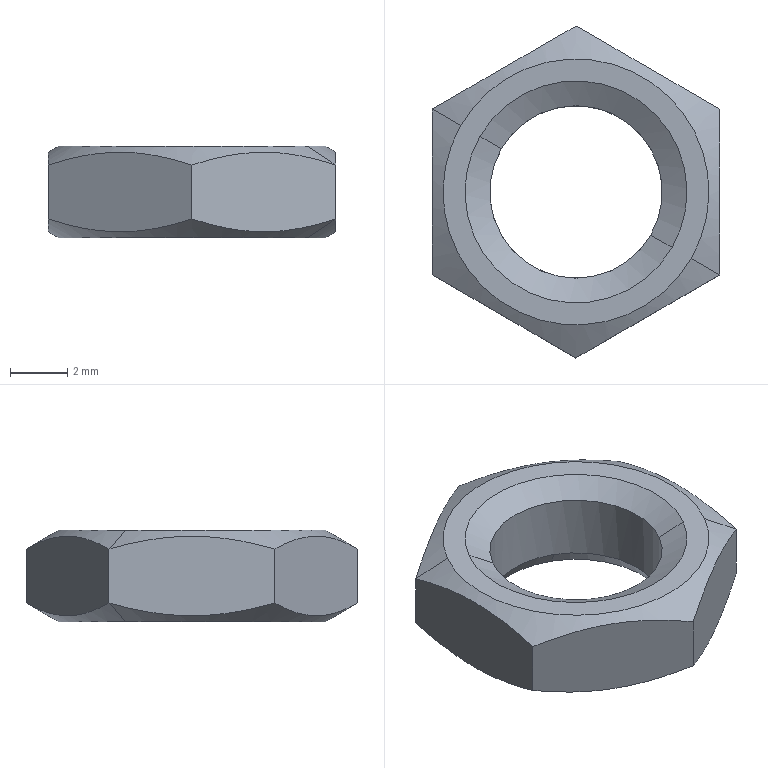Component | SolidWorks | HexThinNutGBT6172.1-M6-1 | 1 solid | 18 faces | box 10 x 11.55 x 3.2 mm | volume 173 mm3 | cone 8 | plane 8 | cylinder 2 | commonest cylinder face diameters 6 x2 | material Purchased Part
STEP:
#1=COLOUR_RGB('',0.7922,0.8196,0.9333);
#2=FILL_AREA_STYLE_COLOUR('',#1);
#3=FILL_AREA_STYLE('',(#2));
#4=SURFACE_STYLE_FILL_AREA(#3);
#5=SURFACE_SIDE_STYLE('',(#4));
#6=SURFACE_STYLE_USAGE(.BOTH.,#5);
#7=PRESENTATION_STYLE_ASSIGNMENT((#6));
#8=CARTESIAN_POINT('',(-1.968,-0.5242,-0.2756));
#9=VERTEX_POINT('',#8);
#10=CARTESIAN_POINT('',(-2.284,-0.3419,-0.2756));
#11=VERTEX_POINT('',#10);
#12=CARTESIAN_POINT('',(-2.126,-0.4331,-0.2756));
#13=DIRECTION('',(0.,0.,1.));
#14=DIRECTION('',(0.8657,-0.5005,0.));
#15=AXIS2_PLACEMENT_3D('',#12,#13,#14);
#16=CIRCLE('',#15,0.1821);
#17=EDGE_CURVE('',#9,#11,#16,.T.);
#18=ORIENTED_EDGE('',*,*,#17,.T.);
#19=CARTESIAN_POINT('',(-2.323,-0.3193,-0.2495));
#20=VERTEX_POINT('',#19);
#21=CARTESIAN_POINT('',(-2.323,-0.3192,-0.2493));
#22=DIRECTION('',(-0.7497,0.4335,0.5));
#23=VECTOR('',#22,39.37);
#24=LINE('',#21,#23);
#25=EDGE_CURVE('',#11,#20,#24,.T.);
#26=ORIENTED_EDGE('',*,*,#25,.T.);
#27=CARTESIAN_POINT('',(-2.126,-0.2058,-0.2495));
#28=VERTEX_POINT('',#27);
#29=CARTESIAN_POINT('',(-2.323,-0.3193,-0.2495));
#30=CARTESIAN_POINT('',(-2.291,-0.3008,-0.2602));
#31=CARTESIAN_POINT('',(-2.258,-0.2819,-0.267));
#32=CARTESIAN_POINT('',(-2.216,-0.2578,-0.2671));
#33=CARTESIAN_POINT('',(-2.208,-0.253,-0.2667));
#34=CARTESIAN_POINT('',(-2.191,-0.2434,-0.2651));
#35=CARTESIAN_POINT('',(-2.183,-0.2386,-0.2639));
#36=CARTESIAN_POINT('',(-2.158,-0.2244,-0.2593));
#37=CARTESIAN_POINT('',(-2.142,-0.215,-0.2548));
#38=CARTESIAN_POINT('',(-2.126,-0.2058,-0.2495));
#39=B_SPLINE_CURVE_WITH_KNOTS('',3,(#29,#30,#31,#32,#33,#34,#35,#36,#37,#38),.UNSPECIFIED.,.F.,.F.,(4,2,2,2,4),(0.,0.002915,0.003644,0.004373,0.005831),.UNSPECIFIED.);
#40=EDGE_CURVE('',#20,#28,#39,.T.);
#41=ORIENTED_EDGE('',*,*,#40,.T.);
#42=CARTESIAN_POINT('',(-1.929,-0.3195,-0.2495));
#43=VERTEX_POINT('',#42);
#44=CARTESIAN_POINT('',(-2.126,-0.2058,-0.2495));
#45=CARTESIAN_POINT('',(-2.094,-0.2243,-0.2602));
#46=CARTESIAN_POINT('',(-2.061,-0.2432,-0.267));
#47=CARTESIAN_POINT('',(-2.019,-0.2674,-0.2671));
#48=CARTESIAN_POINT('',(-2.011,-0.2722,-0.2667));
#49=CARTESIAN_POINT('',(-1.994,-0.2819,-0.2651));
#50=CARTESIAN_POINT('',(-1.986,-0.2866,-0.2639));
#51=CARTESIAN_POINT('',(-1.961,-0.3009,-0.2593));
#52=CARTESIAN_POINT('',(-1.945,-0.3102,-0.2548));
#53=CARTESIAN_POINT('',(-1.929,-0.3195,-0.2495));
#54=B_SPLINE_CURVE_WITH_KNOTS('',3,(#44,#45,#46,#47,#48,#49,#50,#51,#52,#53),.UNSPECIFIED.,.F.,.F.,(4,2,2,2,4),(0.,0.002915,0.003644,0.004373,0.005831),.UNSPECIFIED.);
#55=EDGE_CURVE('',#28,#43,#54,.T.);
#56=ORIENTED_EDGE('',*,*,#55,.T.);
#57=CARTESIAN_POINT('',(-1.929,-0.5468,-0.2495));
#58=VERTEX_POINT('',#57);
#59=CARTESIAN_POINT('',(-1.929,-0.3195,-0.2495));
#60=CARTESIAN_POINT('',(-1.929,-0.3567,-0.2602));
#61=CARTESIAN_POINT('',(-1.929,-0.3943,-0.267));
#62=CARTESIAN_POINT('',(-1.929,-0.4426,-0.2671));
#63=CARTESIAN_POINT('',(-1.929,-0.4523,-0.2667));
#64=CARTESIAN_POINT('',(-1.929,-0.4715,-0.2651));
#65=CARTESIAN_POINT('',(-1.929,-0.4811,-0.2639));
#66=CARTESIAN_POINT('',(-1.929,-0.5095,-0.2593));
#67=CARTESIAN_POINT('',(-1.929,-0.5283,-0.2548));
#68=CARTESIAN_POINT('',(-1.929,-0.5468,-0.2495));
#69=B_SPLINE_CURVE_WITH_KNOTS('',3,(#59,#60,#61,#62,#63,#64,#65,#66,#67,#68),.UNSPECIFIED.,.F.,.F.,(4,2,2,2,4),(0.,0.002915,0.003644,0.004373,0.005831),.UNSPECIFIED.);
#70=EDGE_CURVE('',#43,#58,#69,.T.);
#71=ORIENTED_EDGE('',*,*,#70,.T.);
#72=CARTESIAN_POINT('',(-1.929,-0.547,-0.2493));
#73=DIRECTION('',(0.7497,-0.4335,0.5));
#74=VECTOR('',#73,39.37);
#75=LINE('',#72,#74);
#76=EDGE_CURVE('',#9,#58,#75,.T.);
#77=ORIENTED_EDGE('',*,*,#76,.F.);
#78=EDGE_LOOP('',(#18,#26,#41,#56,#71,#77));
#79=FACE_OUTER_BOUND('',#78,.T.);
#80=CARTESIAN_POINT('',(-2.126,-0.4331,-0.2493));
#81=DIRECTION('',(0.,0.,1.));
#82=DIRECTION('',(0.8657,-0.5005,0.));
#83=AXIS2_PLACEMENT_3D('',#80,#81,#82);
#84=CONICAL_SURFACE('',#83,0.2276,1.047);
#85=ADVANCED_FACE('',(#79),#84,.T.);
#86=CARTESIAN_POINT('',(-2.185,-0.5353,-0.2573));
#87=VERTEX_POINT('',#86);
#88=CARTESIAN_POINT('',(-2.228,-0.374,-0.2573));
#89=VERTEX_POINT('',#88);
#90=CARTESIAN_POINT('',(-2.126,-0.4331,-0.2573));
#91=DIRECTION('',(0.,0.,-1.));
#92=DIRECTION('',(0.5005,0.8657,0.));
#93=AXIS2_PLACEMENT_3D('',#90,#91,#92);
#94=CIRCLE('',#93,0.1181);
#95=EDGE_CURVE('',#87,#89,#94,.T.);
#96=ORIENTED_EDGE('',*,*,#95,.F.);
#97=CARTESIAN_POINT('',(-2.19,-0.5445,-0.2756));
#98=VERTEX_POINT('',#97);
#99=CARTESIAN_POINT('',(-2.187,-0.5391,-0.2649));
#100=DIRECTION('',(-0.2503,-0.4329,-0.866));
#101=VECTOR('',#100,39.37);
#102=LINE('',#99,#101);
#103=EDGE_CURVE('',#87,#98,#102,.T.);
#104=ORIENTED_EDGE('',*,*,#103,.T.);
#105=CARTESIAN_POINT('',(-2.062,-0.3217,-0.2756));
#106=VERTEX_POINT('',#105);
#107=CARTESIAN_POINT('',(-2.126,-0.4331,-0.2756));
#108=DIRECTION('',(0.,0.,-1.));
#109=DIRECTION('',(0.8657,-0.5005,0.));
#110=AXIS2_PLACEMENT_3D('',#107,#108,#109);
#111=CIRCLE('',#110,0.1287);
#112=EDGE_CURVE('',#98,#106,#111,.T.);
#113=ORIENTED_EDGE('',*,*,#112,.T.);
#114=CARTESIAN_POINT('',(-2.067,-0.3308,-0.2573));
#115=VERTEX_POINT('',#114);
#116=CARTESIAN_POINT('',(-2.065,-0.327,-0.2649));
#117=DIRECTION('',(0.2503,0.4329,-0.866));
#118=VECTOR('',#117,39.37);
#119=LINE('',#116,#118);
#120=EDGE_CURVE('',#115,#106,#119,.T.);
#121=ORIENTED_EDGE('',*,*,#120,.F.);
#122=CARTESIAN_POINT('',(-2.126,-0.4331,-0.2573));
#123=DIRECTION('',(0.,0.,-1.));
#124=DIRECTION('',(0.5005,0.8657,0.));
#125=AXIS2_PLACEMENT_3D('',#122,#123,#124);
#126=CIRCLE('',#125,0.1181);
#127=EDGE_CURVE('',#89,#115,#126,.T.);
#128=ORIENTED_EDGE('',*,*,#127,.F.);
#129=EDGE_LOOP('',(#96,#104,#113,#121,#128));
#130=FACE_OUTER_BOUND('',#129,.T.);
#131=CARTESIAN_POINT('',(-2.126,-0.4331,-0.2649));
#132=DIRECTION('',(0.,0.,-1.));
#133=DIRECTION('',(0.5005,0.8657,0.));
#134=AXIS2_PLACEMENT_3D('',#131,#132,#133);
#135=CONICAL_SURFACE('',#134,0.1225,0.5236);
#136=ADVANCED_FACE('',(#130),#135,.F.);
#137=CARTESIAN_POINT('',(-2.024,-0.4922,-0.2573));
#138=VERTEX_POINT('',#137);
#139=CARTESIAN_POINT('',(-2.126,-0.4331,-0.2573));
#140=DIRECTION('',(0.,0.,-1.));
#141=DIRECTION('',(0.5005,0.8657,0.));
#142=AXIS2_PLACEMENT_3D('',#139,#140,#141);
#143=CIRCLE('',#142,0.1181);
#144=EDGE_CURVE('',#138,#87,#143,.T.);
#145=ORIENTED_EDGE('',*,*,#144,.T.);
#146=ORIENTED_EDGE('',*,*,#95,.T.);
#147=CARTESIAN_POINT('',(-2.228,-0.374,-0.1692));
#148=VERTEX_POINT('',#147);
#149=CARTESIAN_POINT('',(-2.228,-0.374,-0.2756));
#150=DIRECTION('',(0.,0.,1.));
#151=VECTOR('',#150,39.37);
#152=LINE('',#149,#151);
#153=EDGE_CURVE('',#89,#148,#152,.T.);
#154=ORIENTED_EDGE('',*,*,#153,.T.);
#155=CARTESIAN_POINT('',(-2.024,-0.4922,-0.1692));
#156=VERTEX_POINT('',#155);
#157=CARTESIAN_POINT('',(-2.126,-0.4331,-0.1692));
#158=DIRECTION('',(0.,0.,-1.));
#159=DIRECTION('',(0.8657,-0.5005,0.));
#160=AXIS2_PLACEMENT_3D('',#157,#158,#159);
#161=CIRCLE('',#160,0.1181);
#162=EDGE_CURVE('',#156,#148,#161,.T.);
#163=ORIENTED_EDGE('',*,*,#162,.F.);
#164=CARTESIAN_POINT('',(-2.024,-0.4922,-0.2756));
#165=DIRECTION('',(0.,0.,1.));
#166=VECTOR('',#165,39.37);
#167=LINE('',#164,#166);
#168=EDGE_CURVE('',#138,#156,#167,.T.);
#169=ORIENTED_EDGE('',*,*,#168,.F.);
#170=EDGE_LOOP('',(#145,#146,#154,#163,#169));
#171=FACE_OUTER_BOUND('',#170,.T.);
#172=CARTESIAN_POINT('',(-2.126,-0.4331,-0.2756));
#173=DIRECTION('',(0.,0.,1.));
#174=DIRECTION('',(0.8657,-0.5005,0.));
#175=AXIS2_PLACEMENT_3D('',#172,#173,#174);
#176=CYLINDRICAL_SURFACE('',#175,0.1181);
#177=ADVANCED_FACE('',(#171),#176,.F.);
#178=CARTESIAN_POINT('',(-2.284,-0.3419,-0.1496));
#179=VERTEX_POINT('',#178);
#180=CARTESIAN_POINT('',(-1.968,-0.5242,-0.1496));
#181=VERTEX_POINT('',#180);
#182=CARTESIAN_POINT('',(-2.126,-0.4331,-0.1496));
#183=DIRECTION('',(0.,0.,-1.));
#184=DIRECTION('',(-0.8657,0.5005,0.));
#185=AXIS2_PLACEMENT_3D('',#182,#183,#184);
#186=CIRCLE('',#185,0.1821);
#187=EDGE_CURVE('',#179,#181,#186,.T.);
#188=ORIENTED_EDGE('',*,*,#187,.T.);
#189=CARTESIAN_POINT('',(-1.929,-0.5468,-0.1757));
#190=VERTEX_POINT('',#189);
#191=CARTESIAN_POINT('',(-1.929,-0.547,-0.1759));
#192=DIRECTION('',(0.7497,-0.4335,-0.5));
#193=VECTOR('',#192,39.37);
#194=LINE('',#191,#193);
#195=EDGE_CURVE('',#181,#190,#194,.T.);
#196=ORIENTED_EDGE('',*,*,#195,.T.);
#197=CARTESIAN_POINT('',(-1.929,-0.3195,-0.1757));
#198=VERTEX_POINT('',#197);
#199=CARTESIAN_POINT('',(-1.929,-0.3195,-0.1757));
#200=CARTESIAN_POINT('',(-1.929,-0.3567,-0.165));
#201=CARTESIAN_POINT('',(-1.929,-0.3943,-0.1582));
#202=CARTESIAN_POINT('',(-1.929,-0.4426,-0.1581));
#203=CARTESIAN_POINT('',(-1.929,-0.4523,-0.1585));
#204=CARTESIAN_POINT('',(-1.929,-0.4715,-0.1601));
#205=CARTESIAN_POINT('',(-1.929,-0.4811,-0.1613));
#206=CARTESIAN_POINT('',(-1.929,-0.5095,-0.1659));
#207=CARTESIAN_POINT('',(-1.929,-0.5283,-0.1703));
#208=CARTESIAN_POINT('',(-1.929,-0.5468,-0.1757));
#209=B_SPLINE_CURVE_WITH_KNOTS('',3,(#199,#200,#201,#202,#203,#204,#205,#206,#207,#208),.UNSPECIFIED.,.F.,.F.,(4,2,2,2,4),(0.,0.002915,0.003644,0.004373,0.005831),.UNSPECIFIED.);
#210=EDGE_CURVE('',#198,#190,#209,.T.);
#211=ORIENTED_EDGE('',*,*,#210,.F.);
#212=CARTESIAN_POINT('',(-2.126,-0.2058,-0.1757));
#213=VERTEX_POINT('',#212);
#214=CARTESIAN_POINT('',(-2.126,-0.2058,-0.1757));
#215=CARTESIAN_POINT('',(-2.094,-0.2243,-0.165));
#216=CARTESIAN_POINT('',(-2.061,-0.2432,-0.1582));
#217=CARTESIAN_POINT('',(-2.019,-0.2674,-0.1581));
#218=CARTESIAN_POINT('',(-2.011,-0.2722,-0.1585));
#219=CARTESIAN_POINT('',(-1.994,-0.2819,-0.1601));
#220=CARTESIAN_POINT('',(-1.986,-0.2866,-0.1613));
#221=CARTESIAN_POINT('',(-1.961,-0.3009,-0.1659));
#222=CARTESIAN_POINT('',(-1.945,-0.3102,-0.1703));
#223=CARTESIAN_POINT('',(-1.929,-0.3195,-0.1757));
#224=B_SPLINE_CURVE_WITH_KNOTS('',3,(#214,#215,#216,#217,#218,#219,#220,#221,#222,#223),.UNSPECIFIED.,.F.,.F.,(4,2,2,2,4),(0.,0.002915,0.003644,0.004373,0.005831),.UNSPECIFIED.);
#225=EDGE_CURVE('',#213,#198,#224,.T.);
#226=ORIENTED_EDGE('',*,*,#225,.F.);
#227=CARTESIAN_POINT('',(-2.323,-0.3193,-0.1757));
#228=VERTEX_POINT('',#227);
#229=CARTESIAN_POINT('',(-2.323,-0.3193,-0.1757));
#230=CARTESIAN_POINT('',(-2.291,-0.3008,-0.165));
#231=CARTESIAN_POINT('',(-2.258,-0.2819,-0.1582));
#232=CARTESIAN_POINT('',(-2.216,-0.2578,-0.1581));
#233=CARTESIAN_POINT('',(-2.208,-0.253,-0.1585));
#234=CARTESIAN_POINT('',(-2.191,-0.2434,-0.1601));
#235=CARTESIAN_POINT('',(-2.183,-0.2386,-0.1613));
#236=CARTESIAN_POINT('',(-2.158,-0.2244,-0.1659));
#237=CARTESIAN_POINT('',(-2.142,-0.215,-0.1703));
#238=CARTESIAN_POINT('',(-2.126,-0.2058,-0.1757));
#239=B_SPLINE_CURVE_WITH_KNOTS('',3,(#229,#230,#231,#232,#233,#234,#235,#236,#237,#238),.UNSPECIFIED.,.F.,.F.,(4,2,2,2,4),(0.,0.002915,0.003644,0.004373,0.005831),.UNSPECIFIED.);
#240=EDGE_CURVE('',#228,#213,#239,.T.);
#241=ORIENTED_EDGE('',*,*,#240,.F.);
#242=CARTESIAN_POINT('',(-2.323,-0.3192,-0.1759));
#243=DIRECTION('',(-0.7497,0.4335,-0.5));
#244=VECTOR('',#243,39.37);
#245=LINE('',#242,#244);
#246=EDGE_CURVE('',#179,#228,#245,.T.);
#247=ORIENTED_EDGE('',*,*,#246,.F.);
#248=EDGE_LOOP('',(#188,#196,#211,#226,#241,#247));
#249=FACE_OUTER_BOUND('',#248,.T.);
#250=CARTESIAN_POINT('',(-2.126,-0.4331,-0.1759));
#251=DIRECTION('',(0.,0.,-1.));
#252=DIRECTION('',(-0.8657,0.5005,0.));
#253=AXIS2_PLACEMENT_3D('',#250,#251,#252);
#254=CONICAL_SURFACE('',#253,0.2276,1.047);
#255=ADVANCED_FACE('',(#249),#254,.T.);
#256=ORIENTED_EDGE('',*,*,#162,.T.);
#257=CARTESIAN_POINT('',(-2.258,-0.357,-0.1496));
#258=VERTEX_POINT('',#257);
#259=CARTESIAN_POINT('',(-2.23,-0.373,-0.1681));
#260=DIRECTION('',(-0.7497,0.4335,0.5));
#261=VECTOR('',#260,39.37);
#262=LINE('',#259,#261);
#263=EDGE_CURVE('',#148,#258,#262,.T.);
#264=ORIENTED_EDGE('',*,*,#263,.T.);
#265=CARTESIAN_POINT('',(-1.994,-0.5092,-0.1496));
#266=VERTEX_POINT('',#265);
#267=CARTESIAN_POINT('',(-2.126,-0.4331,-0.1496));
#268=DIRECTION('',(0.,0.,-1.));
#269=DIRECTION('',(0.8657,-0.5005,0.));
#270=AXIS2_PLACEMENT_3D('',#267,#268,#269);
#271=CIRCLE('',#270,0.152);
#272=EDGE_CURVE('',#266,#258,#271,.T.);
#273=ORIENTED_EDGE('',*,*,#272,.F.);
#274=CARTESIAN_POINT('',(-2.022,-0.4932,-0.1681));
#275=DIRECTION('',(0.7497,-0.4335,0.5));
#276=VECTOR('',#275,39.37);
#277=LINE('',#274,#276);
#278=EDGE_CURVE('',#156,#266,#277,.T.);
#279=ORIENTED_EDGE('',*,*,#278,.F.);
#280=EDGE_LOOP('',(#256,#264,#273,#279));
#281=FACE_OUTER_BOUND('',#280,.T.);
#282=CARTESIAN_POINT('',(-2.126,-0.4331,-0.1681));
#283=DIRECTION('',(0.,0.,1.));
#284=DIRECTION('',(0.8657,-0.5005,0.));
#285=AXIS2_PLACEMENT_3D('',#282,#283,#284);
#286=CONICAL_SURFACE('',#285,0.12,1.047);
#287=ADVANCED_FACE('',(#281),#286,.F.);
#288=ORIENTED_EDGE('',*,*,#17,.F.);
#289=CARTESIAN_POINT('',(-2.126,-0.4331,-0.2756));
#290=DIRECTION('',(0.,0.,1.));
#291=DIRECTION('',(0.8657,-0.5005,0.));
#292=AXIS2_PLACEMENT_3D('',#289,#290,#291);
#293=CIRCLE('',#292,0.1821);
#294=EDGE_CURVE('',#11,#9,#293,.T.);
#295=ORIENTED_EDGE('',*,*,#294,.F.);
#296=EDGE_LOOP('',(#288,#295));
#297=FACE_OUTER_BOUND('',#296,.T.);
#298=CARTESIAN_POINT('',(-2.126,-0.4331,-0.2756));
#299=DIRECTION('',(0.,0.,-1.));
#300=DIRECTION('',(0.8657,-0.5005,0.));
#301=AXIS2_PLACEMENT_3D('',#298,#299,#300);
#302=CIRCLE('',#301,0.1287);
#303=EDGE_CURVE('',#106,#98,#302,.T.);
#304=ORIENTED_EDGE('',*,*,#303,.F.);
#305=ORIENTED_EDGE('',*,*,#112,.F.);
#306=EDGE_LOOP('',(#304,#305));
#307=FACE_BOUND('',#306,.T.);
#308=CARTESIAN_POINT('',(-2.126,-0.6604,-0.2756));
#309=DIRECTION('',(0.,0.,1.));
#310=DIRECTION('',(0.8657,-0.5005,0.));
#311=AXIS2_PLACEMENT_3D('',#308,#309,#310);
#312=PLANE('',#311);
#313=ADVANCED_FACE('',(#297,#307),#312,.F.);
#314=ORIENTED_EDGE('',*,*,#25,.F.);
#315=ORIENTED_EDGE('',*,*,#294,.T.);
#316=ORIENTED_EDGE('',*,*,#76,.T.);
#317=CARTESIAN_POINT('',(-2.126,-0.6604,-0.2495));
#318=VERTEX_POINT('',#317);
#319=CARTESIAN_POINT('',(-1.929,-0.5468,-0.2495));
#320=CARTESIAN_POINT('',(-1.961,-0.5654,-0.2602));
#321=CARTESIAN_POINT('',(-1.994,-0.5842,-0.267));
#322=CARTESIAN_POINT('',(-2.036,-0.6083,-0.2671));
#323=CARTESIAN_POINT('',(-2.044,-0.6132,-0.2667));
#324=CARTESIAN_POINT('',(-2.061,-0.6228,-0.2651));
#325=CARTESIAN_POINT('',(-2.069,-0.6275,-0.2639));
#326=CARTESIAN_POINT('',(-2.094,-0.6417,-0.2593));
#327=CARTESIAN_POINT('',(-2.11,-0.6511,-0.2548));
#328=CARTESIAN_POINT('',(-2.126,-0.6604,-0.2495));
#329=B_SPLINE_CURVE_WITH_KNOTS('',3,(#319,#320,#321,#322,#323,#324,#325,#326,#327,#328),.UNSPECIFIED.,.F.,.F.,(4,2,2,2,4),(0.,0.002915,0.003644,0.004373,0.005831),.UNSPECIFIED.);
#330=EDGE_CURVE('',#58,#318,#329,.T.);
#331=ORIENTED_EDGE('',*,*,#330,.T.);
#332=CARTESIAN_POINT('',(-2.323,-0.5466,-0.2495));
#333=VERTEX_POINT('',#332);
#334=CARTESIAN_POINT('',(-2.126,-0.6604,-0.2495));
#335=CARTESIAN_POINT('',(-2.158,-0.6418,-0.2602));
#336=CARTESIAN_POINT('',(-2.191,-0.6229,-0.267));
#337=CARTESIAN_POINT('',(-2.233,-0.5988,-0.2671));
#338=CARTESIAN_POINT('',(-2.241,-0.5939,-0.2667));
#339=CARTESIAN_POINT('',(-2.258,-0.5843,-0.2651));
#340=CARTESIAN_POINT('',(-2.266,-0.5795,-0.2639));
#341=CARTESIAN_POINT('',(-2.291,-0.5653,-0.2593));
#342=CARTESIAN_POINT('',(-2.307,-0.5559,-0.2548));
#343=CARTESIAN_POINT('',(-2.323,-0.5466,-0.2495));
#344=B_SPLINE_CURVE_WITH_KNOTS('',3,(#334,#335,#336,#337,#338,#339,#340,#341,#342,#343),.UNSPECIFIED.,.F.,.F.,(4,2,2,2,4),(0.,0.002915,0.003644,0.004373,0.005831),.UNSPECIFIED.);
#345=EDGE_CURVE('',#318,#333,#344,.T.);
#346=ORIENTED_EDGE('',*,*,#345,.T.);
#347=CARTESIAN_POINT('',(-2.323,-0.5466,-0.2495));
#348=CARTESIAN_POINT('',(-2.323,-0.5095,-0.2602));
#349=CARTESIAN_POINT('',(-2.323,-0.4718,-0.267));
#350=CARTESIAN_POINT('',(-2.323,-0.4235,-0.2671));
#351=CARTESIAN_POINT('',(-2.323,-0.4138,-0.2667));
#352=CARTESIAN_POINT('',(-2.323,-0.3946,-0.2651));
#353=CARTESIAN_POINT('',(-2.323,-0.3851,-0.2639));
#354=CARTESIAN_POINT('',(-2.323,-0.3566,-0.2593));
#355=CARTESIAN_POINT('',(-2.323,-0.3379,-0.2548));
#356=CARTESIAN_POINT('',(-2.323,-0.3193,-0.2495));
#357=B_SPLINE_CURVE_WITH_KNOTS('',3,(#347,#348,#349,#350,#351,#352,#353,#354,#355,#356),.UNSPECIFIED.,.F.,.F.,(4,2,2,2,4),(0.,0.002915,0.003644,0.004373,0.005831),.UNSPECIFIED.);
#358=EDGE_CURVE('',#333,#20,#357,.T.);
#359=ORIENTED_EDGE('',*,*,#358,.T.);
#360=EDGE_LOOP('',(#314,#315,#316,#331,#346,#359));
#361=FACE_OUTER_BOUND('',#360,.T.);
#362=CARTESIAN_POINT('',(-2.126,-0.4331,-0.2493));
#363=DIRECTION('',(0.,0.,1.));
#364=DIRECTION('',(0.8657,-0.5005,0.));
#365=AXIS2_PLACEMENT_3D('',#362,#363,#364);
#366=CONICAL_SURFACE('',#365,0.2276,1.047);
#367=ADVANCED_FACE('',(#361),#366,.T.);
#368=ORIENTED_EDGE('',*,*,#103,.F.);
#369=ORIENTED_EDGE('',*,*,#144,.F.);
#370=CARTESIAN_POINT('',(-2.126,-0.4331,-0.2573));
#371=DIRECTION('',(0.,0.,-1.));
#372=DIRECTION('',(0.5005,0.8657,0.));
#373=AXIS2_PLACEMENT_3D('',#370,#371,#372);
#374=CIRCLE('',#373,0.1181);
#375=EDGE_CURVE('',#115,#138,#374,.T.);
#376=ORIENTED_EDGE('',*,*,#375,.F.);
#377=ORIENTED_EDGE('',*,*,#120,.T.);
#378=ORIENTED_EDGE('',*,*,#303,.T.);
#379=EDGE_LOOP('',(#368,#369,#376,#377,#378));
#380=FACE_OUTER_BOUND('',#379,.T.);
#381=CARTESIAN_POINT('',(-2.126,-0.4331,-0.2649));
#382=DIRECTION('',(0.,0.,-1.));
#383=DIRECTION('',(0.5005,0.8657,0.));
#384=AXIS2_PLACEMENT_3D('',#381,#382,#383);
#385=CONICAL_SURFACE('',#384,0.1225,0.5236);
#386=ADVANCED_FACE('',(#380),#385,.F.);
#387=ORIENTED_EDGE('',*,*,#358,.F.);
#388=CARTESIAN_POINT('',(-2.323,-0.5466,-0.1757));
#389=VERTEX_POINT('',#388);
#390=CARTESIAN_POINT('',(-2.323,-0.5466,-0.2756));
#391=DIRECTION('',(0.,0.,1.));
#392=VECTOR('',#391,39.37);
#393=LINE('',#390,#392);
#394=EDGE_CURVE('',#333,#389,#393,.T.);
#395=ORIENTED_EDGE('',*,*,#394,.T.);
#396=CARTESIAN_POINT('',(-2.323,-0.5466,-0.1757));
#397=CARTESIAN_POINT('',(-2.323,-0.5095,-0.165));
#398=CARTESIAN_POINT('',(-2.323,-0.4718,-0.1582));
#399=CARTESIAN_POINT('',(-2.323,-0.4235,-0.1581));
#400=CARTESIAN_POINT('',(-2.323,-0.4138,-0.1585));
#401=CARTESIAN_POINT('',(-2.323,-0.3946,-0.1601));
#402=CARTESIAN_POINT('',(-2.323,-0.3851,-0.1613));
#403=CARTESIAN_POINT('',(-2.323,-0.3566,-0.1659));
#404=CARTESIAN_POINT('',(-2.323,-0.3379,-0.1703));
#405=CARTESIAN_POINT('',(-2.323,-0.3193,-0.1757));
#406=B_SPLINE_CURVE_WITH_KNOTS('',3,(#396,#397,#398,#399,#400,#401,#402,#403,#404,#405),.UNSPECIFIED.,.F.,.F.,(4,2,2,2,4),(0.,0.002915,0.003644,0.004373,0.005831),.UNSPECIFIED.);
#407=EDGE_CURVE('',#389,#228,#406,.T.);
#408=ORIENTED_EDGE('',*,*,#407,.T.);
#409=CARTESIAN_POINT('',(-2.323,-0.3193,-0.2756));
#410=DIRECTION('',(0.,0.,-1.));
#411=VECTOR('',#410,39.37);
#412=LINE('',#409,#411);
#413=EDGE_CURVE('',#228,#20,#412,.T.);
#414=ORIENTED_EDGE('',*,*,#413,.T.);
#415=EDGE_LOOP('',(#387,#395,#408,#414));
#416=FACE_OUTER_BOUND('',#415,.T.);
#417=CARTESIAN_POINT('',(-2.323,-0.3193,-0.2756));
#418=DIRECTION('',(-1.,0.0006061,0.));
#419=DIRECTION('',(-0.0006061,-1.,0.));
#420=AXIS2_PLACEMENT_3D('',#417,#418,#419);
#421=PLANE('',#420);
#422=ADVANCED_FACE('',(#416),#421,.T.);
#423=ORIENTED_EDGE('',*,*,#345,.F.);
#424=CARTESIAN_POINT('',(-2.126,-0.6604,-0.1757));
#425=VERTEX_POINT('',#424);
#426=CARTESIAN_POINT('',(-2.126,-0.6604,-0.2756));
#427=DIRECTION('',(0.,0.,1.));
#428=VECTOR('',#427,39.37);
#429=LINE('',#426,#428);
#430=EDGE_CURVE('',#318,#425,#429,.T.);
#431=ORIENTED_EDGE('',*,*,#430,.T.);
#432=CARTESIAN_POINT('',(-2.126,-0.6604,-0.1757));
#433=CARTESIAN_POINT('',(-2.158,-0.6418,-0.165));
#434=CARTESIAN_POINT('',(-2.191,-0.6229,-0.1582));
#435=CARTESIAN_POINT('',(-2.233,-0.5988,-0.1581));
#436=CARTESIAN_POINT('',(-2.241,-0.5939,-0.1585));
#437=CARTESIAN_POINT('',(-2.258,-0.5843,-0.1601));
#438=CARTESIAN_POINT('',(-2.266,-0.5795,-0.1613));
#439=CARTESIAN_POINT('',(-2.291,-0.5653,-0.1659));
#440=CARTESIAN_POINT('',(-2.307,-0.5559,-0.1703));
#441=CARTESIAN_POINT('',(-2.323,-0.5466,-0.1757));
#442=B_SPLINE_CURVE_WITH_KNOTS('',3,(#432,#433,#434,#435,#436,#437,#438,#439,#440,#441),.UNSPECIFIED.,.F.,.F.,(4,2,2,2,4),(0.,0.002915,0.003644,0.004373,0.005831),.UNSPECIFIED.);
#443=EDGE_CURVE('',#425,#389,#442,.T.);
#444=ORIENTED_EDGE('',*,*,#443,.T.);
#445=ORIENTED_EDGE('',*,*,#394,.F.);
#446=EDGE_LOOP('',(#423,#431,#444,#445));
#447=FACE_OUTER_BOUND('',#446,.T.);
#448=CARTESIAN_POINT('',(-2.323,-0.5466,-0.2756));
#449=DIRECTION('',(-0.5005,-0.8657,0.));
#450=DIRECTION('',(0.,0.,-1.));
#451=AXIS2_PLACEMENT_3D('',#448,#449,#450);
#452=PLANE('',#451);
#453=ADVANCED_FACE('',(#447),#452,.T.);
#454=ORIENTED_EDGE('',*,*,#330,.F.);
#455=CARTESIAN_POINT('',(-1.929,-0.5468,-0.2756));
#456=DIRECTION('',(0.,0.,1.));
#457=VECTOR('',#456,39.37);
#458=LINE('',#455,#457);
#459=EDGE_CURVE('',#58,#190,#458,.T.);
#460=ORIENTED_EDGE('',*,*,#459,.T.);
#461=CARTESIAN_POINT('',(-1.929,-0.5468,-0.1757));
#462=CARTESIAN_POINT('',(-1.961,-0.5654,-0.165));
#463=CARTESIAN_POINT('',(-1.994,-0.5842,-0.1582));
#464=CARTESIAN_POINT('',(-2.036,-0.6083,-0.1581));
#465=CARTESIAN_POINT('',(-2.044,-0.6132,-0.1585));
#466=CARTESIAN_POINT('',(-2.061,-0.6228,-0.1601));
#467=CARTESIAN_POINT('',(-2.069,-0.6275,-0.1613));
#468=CARTESIAN_POINT('',(-2.094,-0.6417,-0.1659));
#469=CARTESIAN_POINT('',(-2.11,-0.6511,-0.1703));
#470=CARTESIAN_POINT('',(-2.126,-0.6604,-0.1757));
#471=B_SPLINE_CURVE_WITH_KNOTS('',3,(#461,#462,#463,#464,#465,#466,#467,#468,#469,#470),.UNSPECIFIED.,.F.,.F.,(4,2,2,2,4),(0.,0.002915,0.003644,0.004373,0.005831),.UNSPECIFIED.);
#472=EDGE_CURVE('',#190,#425,#471,.T.);
#473=ORIENTED_EDGE('',*,*,#472,.T.);
#474=ORIENTED_EDGE('',*,*,#430,.F.);
#475=EDGE_LOOP('',(#454,#460,#473,#474));
#476=FACE_OUTER_BOUND('',#475,.T.);
#477=CARTESIAN_POINT('',(-2.126,-0.6604,-0.2756));
#478=DIRECTION('',(0.4995,-0.8663,0.));
#479=DIRECTION('',(0.8663,0.4995,0.));
#480=AXIS2_PLACEMENT_3D('',#477,#478,#479);
#481=PLANE('',#480);
#482=ADVANCED_FACE('',(#476),#481,.T.);
#483=ORIENTED_EDGE('',*,*,#70,.F.);
#484=CARTESIAN_POINT('',(-1.929,-0.3195,-0.2756));
#485=DIRECTION('',(0.,0.,1.));
#486=VECTOR('',#485,39.37);
#487=LINE('',#484,#486);
#488=EDGE_CURVE('',#43,#198,#487,.T.);
#489=ORIENTED_EDGE('',*,*,#488,.T.);
#490=ORIENTED_EDGE('',*,*,#210,.T.);
#491=ORIENTED_EDGE('',*,*,#459,.F.);
#492=EDGE_LOOP('',(#483,#489,#490,#491));
#493=FACE_OUTER_BOUND('',#492,.T.);
#494=CARTESIAN_POINT('',(-1.929,-0.5468,-0.2756));
#495=DIRECTION('',(1.,-0.0006061,0.));
#496=DIRECTION('',(0.0006061,1.,0.));
#497=AXIS2_PLACEMENT_3D('',#494,#495,#496);
#498=PLANE('',#497);
#499=ADVANCED_FACE('',(#493),#498,.T.);
#500=ORIENTED_EDGE('',*,*,#55,.F.);
#501=CARTESIAN_POINT('',(-2.126,-0.2058,-0.2756));
#502=DIRECTION('',(0.,0.,1.));
#503=VECTOR('',#502,39.37);
#504=LINE('',#501,#503);
#505=EDGE_CURVE('',#28,#213,#504,.T.);
#506=ORIENTED_EDGE('',*,*,#505,.T.);
#507=ORIENTED_EDGE('',*,*,#225,.T.);
#508=ORIENTED_EDGE('',*,*,#488,.F.);
#509=EDGE_LOOP('',(#500,#506,#507,#508));
#510=FACE_OUTER_BOUND('',#509,.T.);
#511=CARTESIAN_POINT('',(-1.929,-0.3195,-0.2756));
#512=DIRECTION('',(0.5005,0.8657,0.));
#513=DIRECTION('',(0.,0.,1.));
#514=AXIS2_PLACEMENT_3D('',#511,#512,#513);
#515=PLANE('',#514);
#516=ADVANCED_FACE('',(#510),#515,.T.);
#517=ORIENTED_EDGE('',*,*,#40,.F.);
#518=ORIENTED_EDGE('',*,*,#413,.F.);
#519=ORIENTED_EDGE('',*,*,#240,.T.);
#520=ORIENTED_EDGE('',*,*,#505,.F.);
#521=EDGE_LOOP('',(#517,#518,#519,#520));
#522=FACE_OUTER_BOUND('',#521,.T.);
#523=CARTESIAN_POINT('',(-2.126,-0.2058,-0.2756));
#524=DIRECTION('',(-0.4995,0.8663,0.));
#525=DIRECTION('',(-0.8663,-0.4995,0.));
#526=AXIS2_PLACEMENT_3D('',#523,#524,#525);
#527=PLANE('',#526);
#528=ADVANCED_FACE('',(#522),#527,.T.);
#529=ORIENTED_EDGE('',*,*,#153,.F.);
#530=ORIENTED_EDGE('',*,*,#127,.T.);
#531=ORIENTED_EDGE('',*,*,#375,.T.);
#532=ORIENTED_EDGE('',*,*,#168,.T.);
#533=CARTESIAN_POINT('',(-2.126,-0.4331,-0.1692));
#534=DIRECTION('',(0.,0.,-1.));
#535=DIRECTION('',(0.8657,-0.5005,0.));
#536=AXIS2_PLACEMENT_3D('',#533,#534,#535);
#537=CIRCLE('',#536,0.1181);
#538=EDGE_CURVE('',#148,#156,#537,.T.);
#539=ORIENTED_EDGE('',*,*,#538,.F.);
#540=EDGE_LOOP('',(#529,#530,#531,#532,#539));
#541=FACE_OUTER_BOUND('',#540,.T.);
#542=CARTESIAN_POINT('',(-2.126,-0.4331,-0.2756));
#543=DIRECTION('',(0.,0.,1.));
#544=DIRECTION('',(0.8657,-0.5005,0.));
#545=AXIS2_PLACEMENT_3D('',#542,#543,#544);
#546=CYLINDRICAL_SURFACE('',#545,0.1181);
#547=ADVANCED_FACE('',(#541),#546,.F.);
#548=ORIENTED_EDGE('',*,*,#195,.F.);
#549=CARTESIAN_POINT('',(-2.126,-0.4331,-0.1496));
#550=DIRECTION('',(0.,0.,-1.));
#551=DIRECTION('',(-0.8657,0.5005,0.));
#552=AXIS2_PLACEMENT_3D('',#549,#550,#551);
#553=CIRCLE('',#552,0.1821);
#554=EDGE_CURVE('',#181,#179,#553,.T.);
#555=ORIENTED_EDGE('',*,*,#554,.T.);
#556=ORIENTED_EDGE('',*,*,#246,.T.);
#557=ORIENTED_EDGE('',*,*,#407,.F.);
#558=ORIENTED_EDGE('',*,*,#443,.F.);
#559=ORIENTED_EDGE('',*,*,#472,.F.);
#560=EDGE_LOOP('',(#548,#555,#556,#557,#558,#559));
#561=FACE_OUTER_BOUND('',#560,.T.);
#562=CARTESIAN_POINT('',(-2.126,-0.4331,-0.1759));
#563=DIRECTION('',(0.,0.,-1.));
#564=DIRECTION('',(-0.8657,0.5005,0.));
#565=AXIS2_PLACEMENT_3D('',#562,#563,#564);
#566=CONICAL_SURFACE('',#565,0.2276,1.047);
#567=ADVANCED_FACE('',(#561),#566,.T.);
#568=ORIENTED_EDGE('',*,*,#263,.F.);
#569=ORIENTED_EDGE('',*,*,#538,.T.);
#570=ORIENTED_EDGE('',*,*,#278,.T.);
#571=CARTESIAN_POINT('',(-2.126,-0.4331,-0.1496));
#572=DIRECTION('',(0.,0.,-1.));
#573=DIRECTION('',(0.8657,-0.5005,0.));
#574=AXIS2_PLACEMENT_3D('',#571,#572,#573);
#575=CIRCLE('',#574,0.152);
#576=EDGE_CURVE('',#258,#266,#575,.T.);
#577=ORIENTED_EDGE('',*,*,#576,.F.);
#578=EDGE_LOOP('',(#568,#569,#570,#577));
#579=FACE_OUTER_BOUND('',#578,.T.);
#580=CARTESIAN_POINT('',(-2.126,-0.4331,-0.1681));
#581=DIRECTION('',(0.,0.,1.));
#582=DIRECTION('',(0.8657,-0.5005,0.));
#583=AXIS2_PLACEMENT_3D('',#580,#581,#582);
#584=CONICAL_SURFACE('',#583,0.12,1.047);
#585=ADVANCED_FACE('',(#579),#584,.F.);
#586=ORIENTED_EDGE('',*,*,#187,.F.);
#587=ORIENTED_EDGE('',*,*,#554,.F.);
#588=EDGE_LOOP('',(#586,#587));
#589=FACE_OUTER_BOUND('',#588,.T.);
#590=ORIENTED_EDGE('',*,*,#272,.T.);
#591=ORIENTED_EDGE('',*,*,#576,.T.);
#592=EDGE_LOOP('',(#590,#591));
#593=FACE_BOUND('',#592,.T.);
#594=CARTESIAN_POINT('',(-2.126,-0.6604,-0.1496));
#595=DIRECTION('',(0.,0.,1.));
#596=DIRECTION('',(0.8657,-0.5005,0.));
#597=AXIS2_PLACEMENT_3D('',#594,#595,#596);
#598=PLANE('',#597);
#599=ADVANCED_FACE('',(#589,#593),#598,.T.);
#600=CLOSED_SHELL('',(#85,#136,#177,#255,#287,#313,#367,#386,#422,#453,#482,#499,#516,#528,#547,#567,#585,#599));
#601=MANIFOLD_SOLID_BREP('',#600);
#602=STYLED_ITEM('',(#7),#601);
#603=PRESENTATION_LAYER_ASSIGNMENT('','',(#602));
#604=CARTESIAN_POINT('',(0.,0.,0.));
#605=DIRECTION('',(0.,0.,1.));
#606=DIRECTION('',(1.,0.,0.));
#607=AXIS2_PLACEMENT_3D('',#604,#605,#606);
#608=(LENGTH_UNIT()NAMED_UNIT(*)SI_UNIT($,.METRE.));
#609=LENGTH_MEASURE_WITH_UNIT(LENGTH_MEASURE(0.0254),#608);
#610=DIMENSIONAL_EXPONENTS(1.,0.,0.,0.,0.,0.,0.);
#611=(CONVERSION_BASED_UNIT('',#609)LENGTH_UNIT()NAMED_UNIT(#610));
#612=UNCERTAINTY_MEASURE_WITH_UNIT(LENGTH_MEASURE(0.00001),#611,'','');
#613=(NAMED_UNIT(*)PLANE_ANGLE_UNIT()SI_UNIT($,.RADIAN.));
#614=(NAMED_UNIT(*)SI_UNIT($,.STERADIAN.)SOLID_ANGLE_UNIT());
#615=(GEOMETRIC_REPRESENTATION_CONTEXT(3)GLOBAL_UNCERTAINTY_ASSIGNED_CONTEXT((#612))GLOBAL_UNIT_ASSIGNED_CONTEXT((#611,#613,#614))REPRESENTATION_CONTEXT('',''));
#616=ADVANCED_BREP_SHAPE_REPRESENTATION('',(#601,#607),#615);
#617=(LENGTH_UNIT()NAMED_UNIT(*)SI_UNIT($,.METRE.));
#618=LENGTH_MEASURE_WITH_UNIT(LENGTH_MEASURE(0.0254),#617);
#619=DIMENSIONAL_EXPONENTS(1.,0.,0.,0.,0.,0.,0.);
#620=(CONVERSION_BASED_UNIT('',#618)LENGTH_UNIT()NAMED_UNIT(#619));
#621=UNCERTAINTY_MEASURE_WITH_UNIT(LENGTH_MEASURE(0.00001),#620,'','');
#622=(NAMED_UNIT(*)PLANE_ANGLE_UNIT()SI_UNIT($,.RADIAN.));
#623=(NAMED_UNIT(*)SI_UNIT($,.STERADIAN.)SOLID_ANGLE_UNIT());
#624=(GEOMETRIC_REPRESENTATION_CONTEXT(3)GLOBAL_UNCERTAINTY_ASSIGNED_CONTEXT((#621))GLOBAL_UNIT_ASSIGNED_CONTEXT((#620,#622,#623))REPRESENTATION_CONTEXT('',''));
#625=MECHANICAL_DESIGN_GEOMETRIC_PRESENTATION_REPRESENTATION('',(#602),#624);